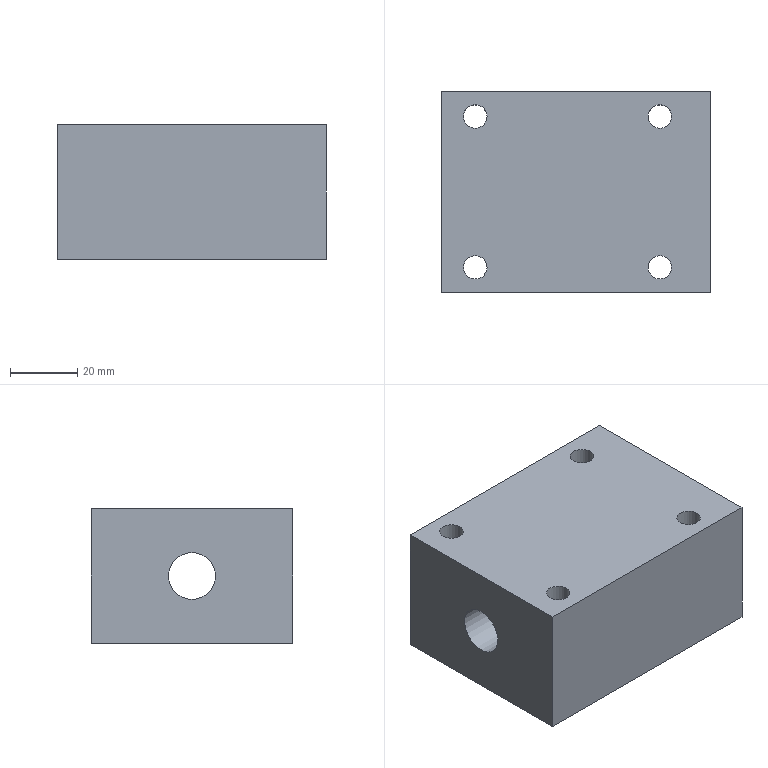Component | NX | VALVE_BODY | 1 solid | 19 faces | volume 148184 mm3 | cylinder 10 | plane 9 | commonest cylinder face diameters 7 x4 5 x2 26.6 x1 19.2 x1 14 x1 30 x1